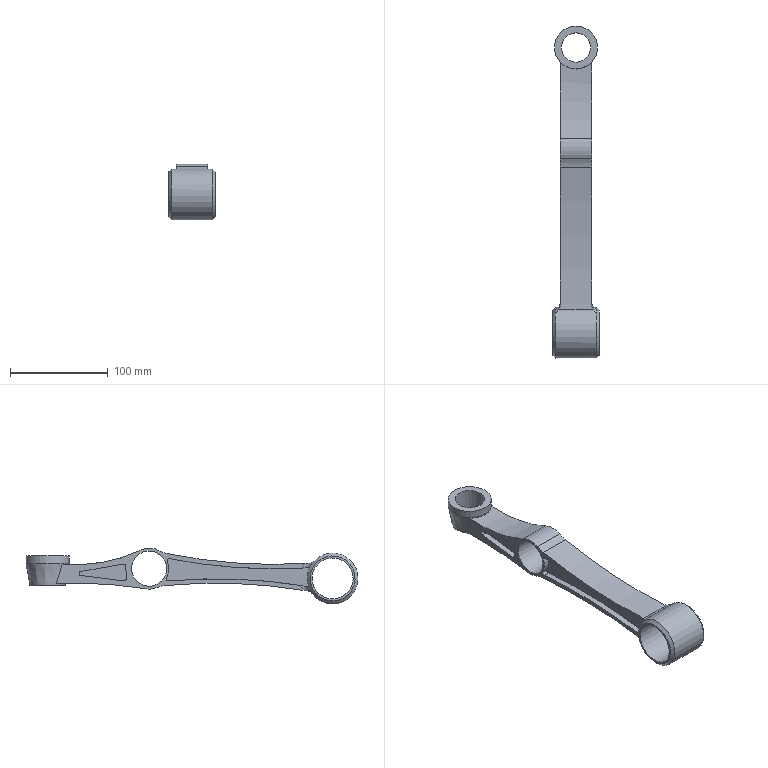Component | NX | BSMP3JX11L_3D | 1 solid | 57 faces | volume 194731 mm3 | cylinder 33 | plane 16 | torus 4 | cone 3 | spline 1 | commonest cylinder face diameters 4 x10 1112.899 x4 42 x3 52 x3 1103.899 x2 60 x2 14 x2 40 x2